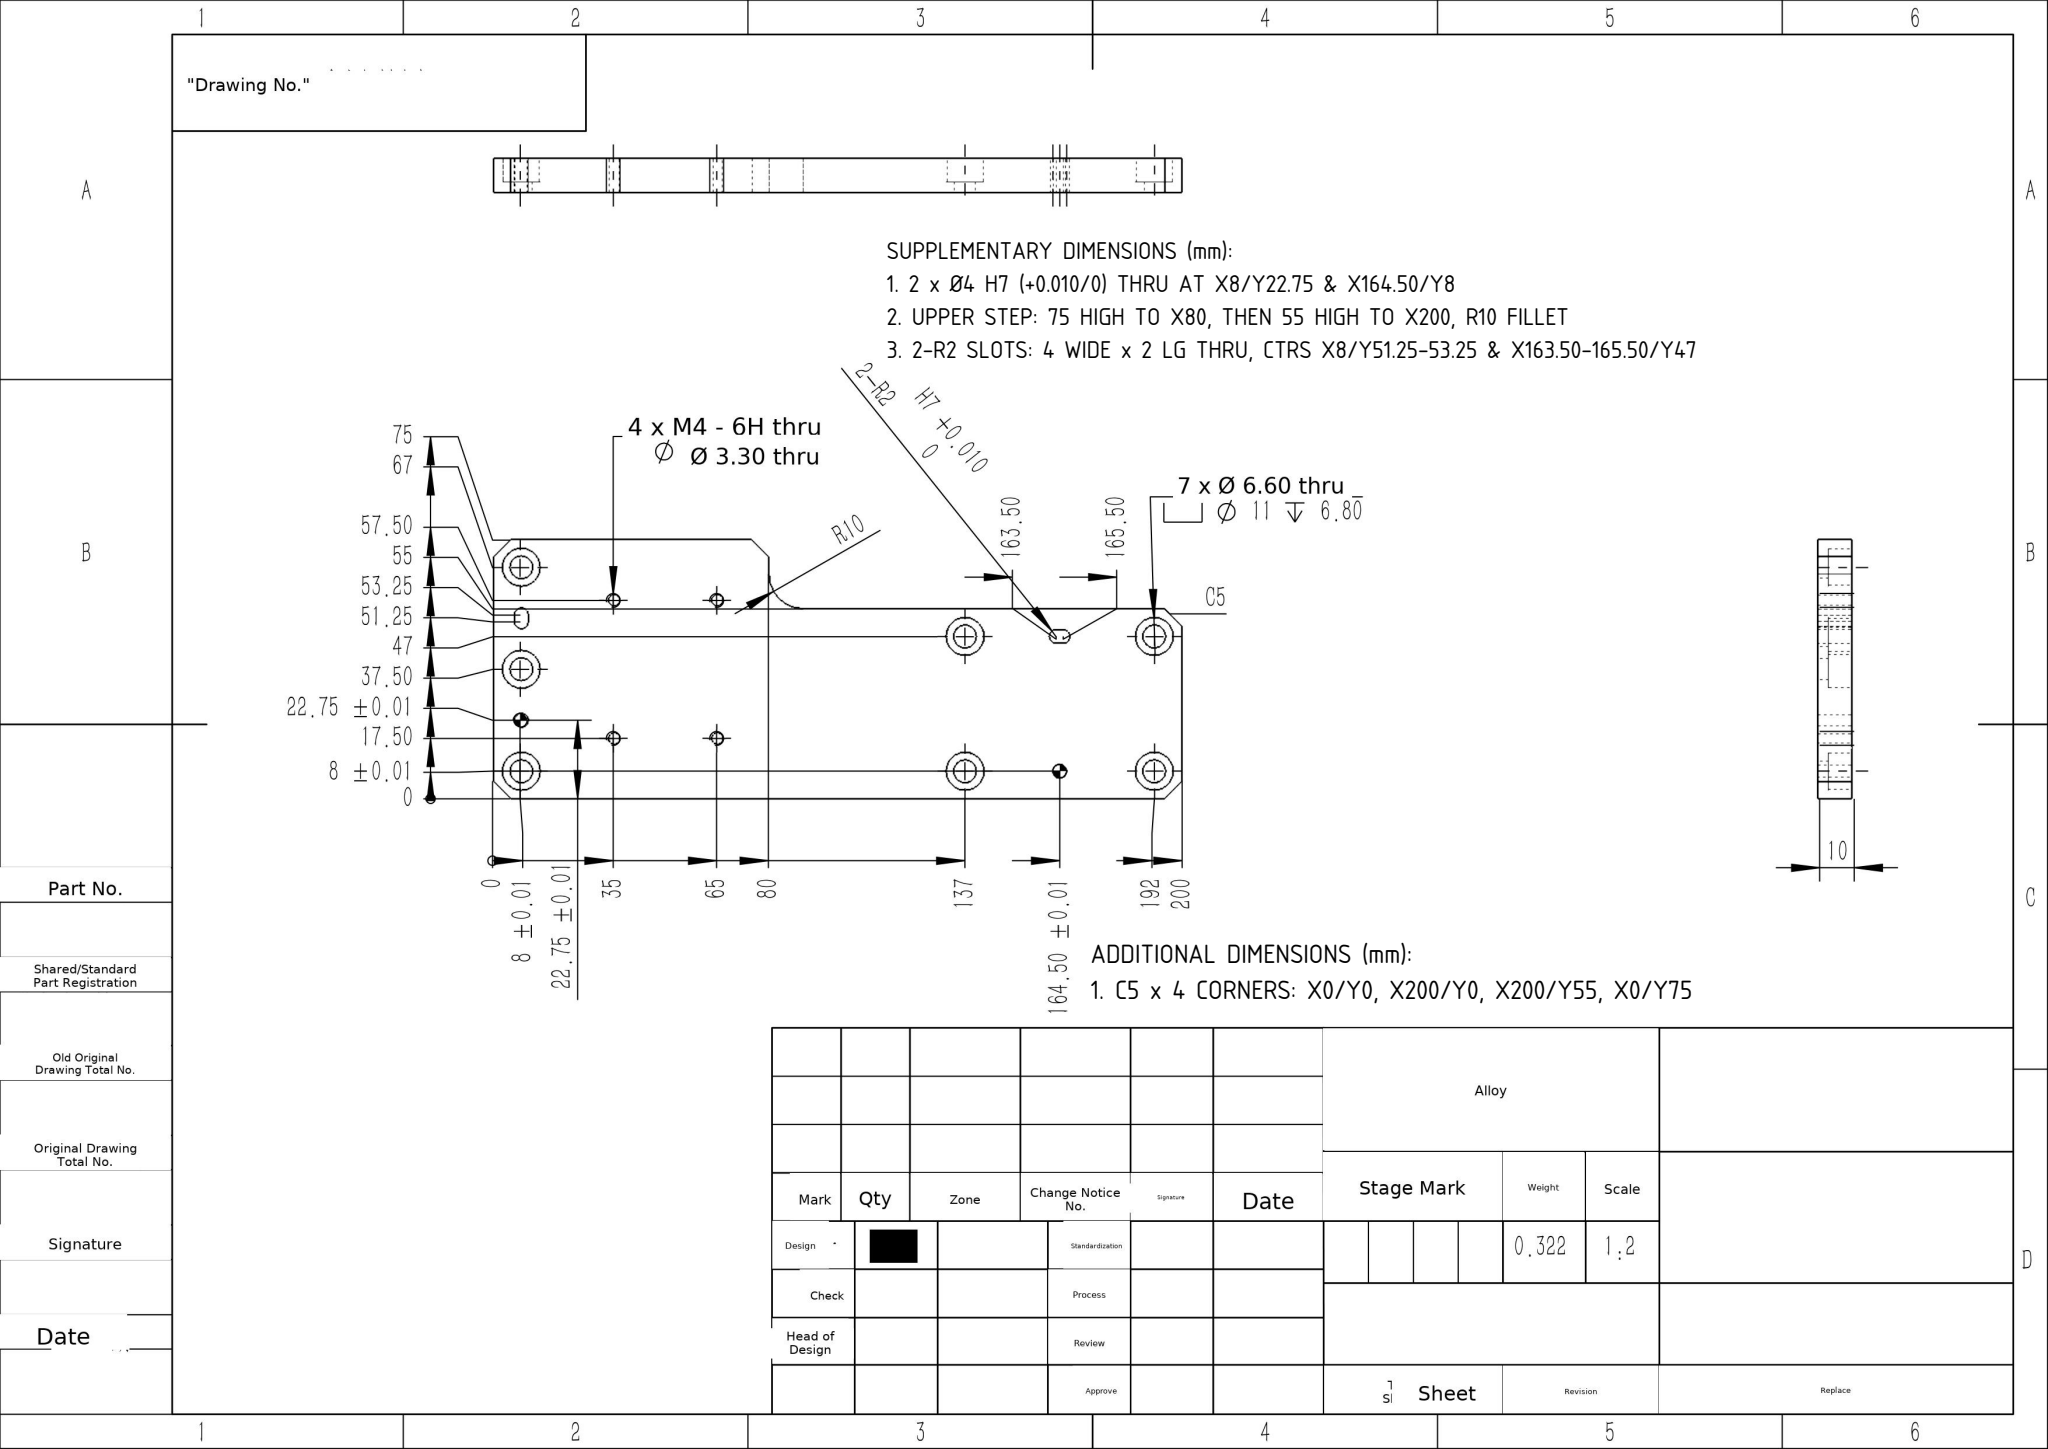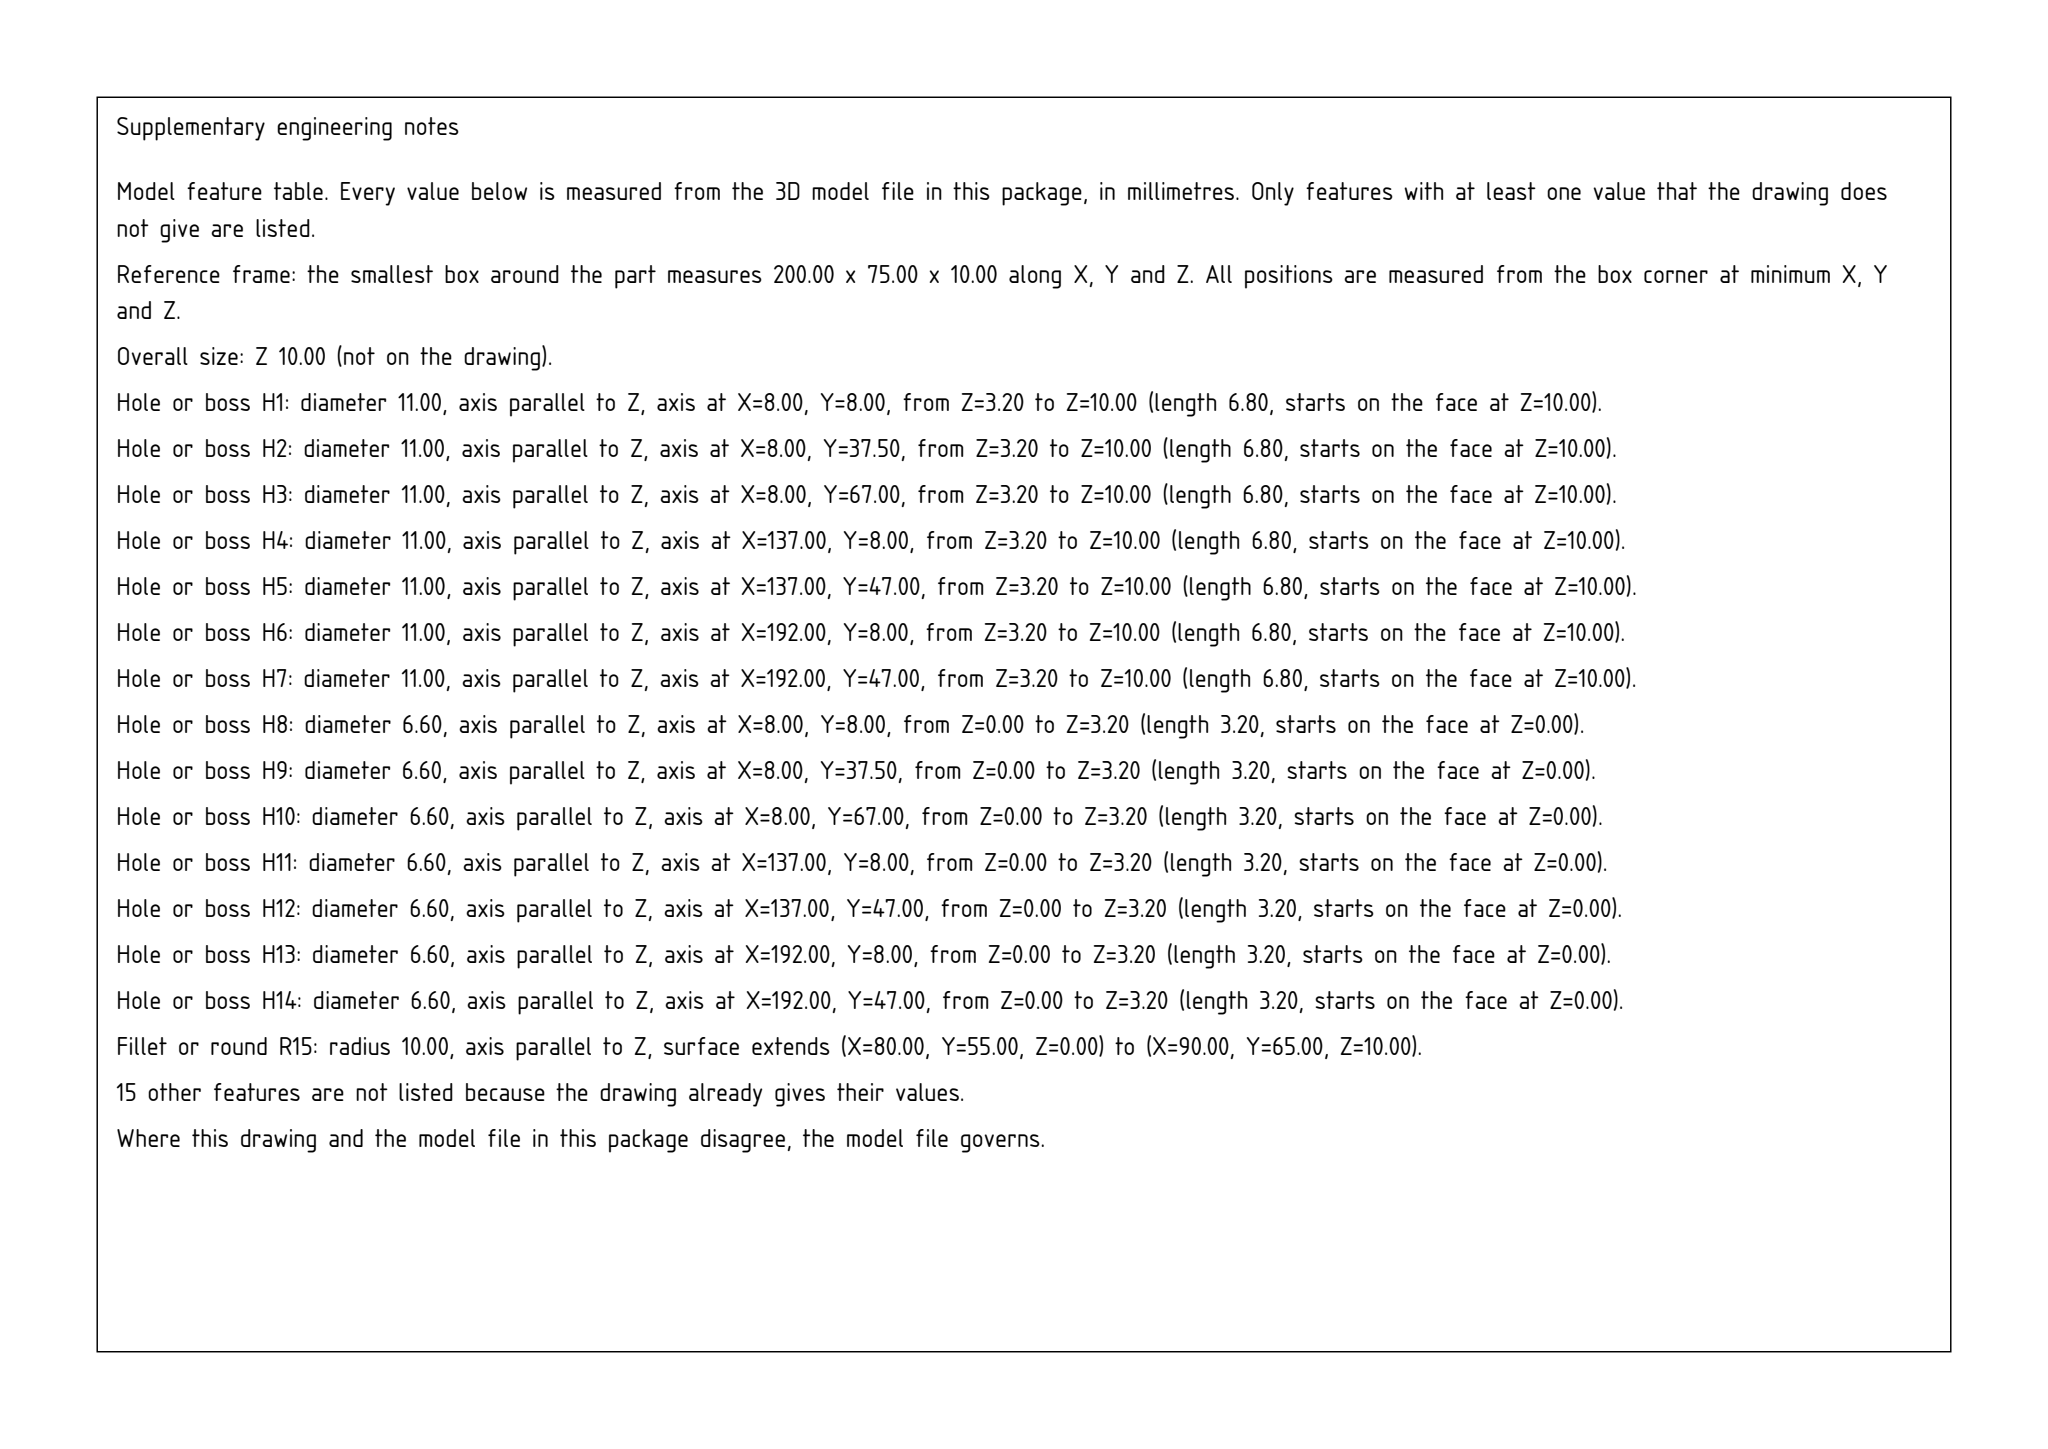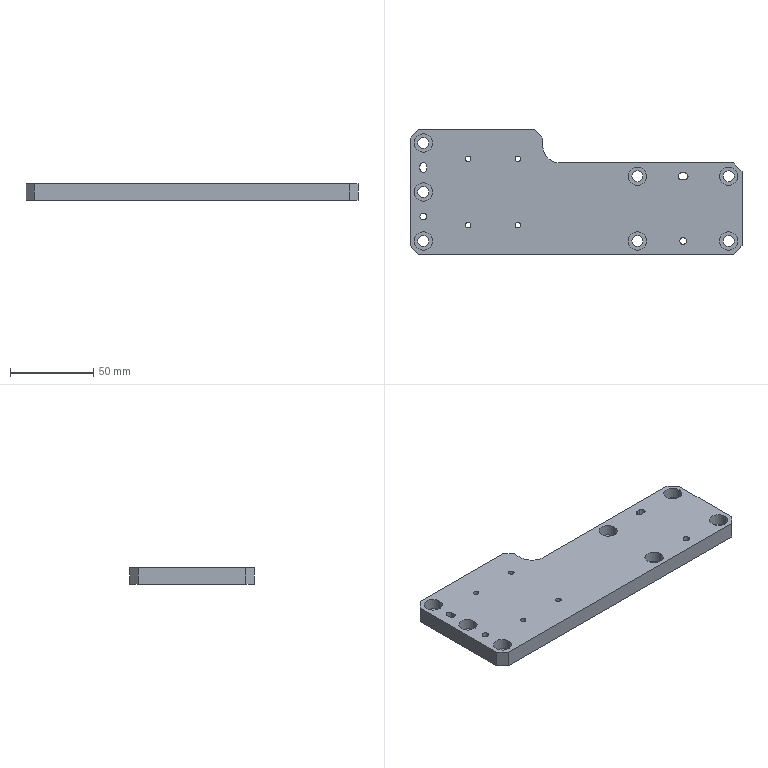Part | SolidWorks | mm | 1 solid | 70 faces | box 200 x 75 x 10 mm | volume 119295 mm3 | cylinder 46 | plane 24 | commonest cylinder face diameters 11 x14 6.6 x14 4 x9 3.3 x8 20 x1
build123d program:
from build123d import *

# Parameters (mm, degrees)
SKETCH1_W                                       = 200
SKETCH1_H                                       = 75
BOSS_EXTRUDE1_DEPTH                             = 5
SKETCH2_W                                       = 120
SKETCH2_H                                       = 20
CUT_EXTRUDE1_DEPTH                              = 108.267
M6_HEX_SOCKET_HEAD_CAP_SCREW_CBORE1_D           = 6.6
M6_HEX_SOCKET_HEAD_CAP_SCREW_CBORE1_CBORE_D     = 11
M6_HEX_SOCKET_HEAD_CAP_SCREW_CBORE1_CBORE_DEPTH = 6.8
F_4_0MM_DOWEL_PIN_HOLE1_D                       = 4
M4_TAPPED_HOLE1_D                               = 3.3
CUT_EXTRUDE2_DEPTH                              = 108.267
CHAMFER1_SIZE                                   = 5
FILLET1_R                                       = 10


with BuildPart() as part:
    # Sketch1 → Boss-Extrude1 (new, symmetric)
    with BuildSketch(Plane.XY):
        Rectangle(SKETCH1_W, SKETCH1_H)
    extrude(amount=BOSS_EXTRUDE1_DEPTH, both=True)

    # Sketch2 → Cut-Extrude1 (cut, through all)
    with BuildSketch(Plane.XY.offset(5)):
        with Locations((40, 27.5)):
            Rectangle(SKETCH2_W, SKETCH2_H)
    extrude(amount=-CUT_EXTRUDE1_DEPTH, mode=Mode.SUBTRACT)

    # M6 Hex Socket Head Cap Screw CBORE1 (through all)
    with Locations(Plane.XY.offset(5)):
        with Locations((-92, 29.5), (-92, 0), (-92, -29.5), (92, 9.5), (92, -29.5), (37, 9.5), (37, -29.5)):
            CounterBoreHole(M6_HEX_SOCKET_HEAD_CAP_SCREW_CBORE1_D / 2, M6_HEX_SOCKET_HEAD_CAP_SCREW_CBORE1_CBORE_D / 2, M6_HEX_SOCKET_HEAD_CAP_SCREW_CBORE1_CBORE_DEPTH)

    # 4.0mm Dowel Pin Hole1 (through all)
    with Locations(Plane.XY.offset(5)):
        with Locations((-92, 14.75), (-92, -14.75), (64.5, 9.5), (64.5, -29.5)):
            Hole(F_4_0MM_DOWEL_PIN_HOLE1_D / 2)

    # M4 Tapped Hole1 (through all)
    with Locations(Plane.XY.offset(5)):
        with Locations((-65, 20), (-35, 20), (-65, -20), (-35, -20)):
            Hole(M4_TAPPED_HOLE1_D / 2)

    # Sketch9 → Cut-Extrude2 (cut, through all)
    with BuildSketch(Plane.XY.offset(5)):
        with BuildLine():
            Line((-90, 15.75), (-90, 13.75))
            ThreePointArc((-90, 13.75), (-92, 11.75), (-94, 13.75))
            Line((-94, 13.75), (-94, 15.75))
            ThreePointArc((-94, 15.75), (-92, 17.75), (-90, 15.75))
        make_face()
        with BuildLine():
            Line((63.5, 11.5), (65.5, 11.5))
            ThreePointArc((65.5, 11.5), (67.5, 9.5), (65.5, 7.5))
            Line((65.5, 7.5), (63.5, 7.5))
            ThreePointArc((63.5, 7.5), (61.5, 9.5), (63.5, 11.5))
        make_face()
    extrude(amount=-CUT_EXTRUDE2_DEPTH, mode=Mode.SUBTRACT)

    # Chamfer1
    chamfer1_edges = [part.edges().sort_by_distance(p)[0] for p in [
        (-20, 37.5, 0),
        (100, 17.5, 0),
        (100, -37.5, 0),
        (-100, -37.5, 0),
        (-100, 37.5, 0),
    ]]
    chamfer(chamfer1_edges, length=CHAMFER1_SIZE)

    # Fillet1
    fillet1_edges = [part.edges().sort_by_distance(p)[0] for p in [
        (-20, 17.5, 0),
    ]]
    fillet(fillet1_edges, radius=FILLET1_R)


solid = part.part